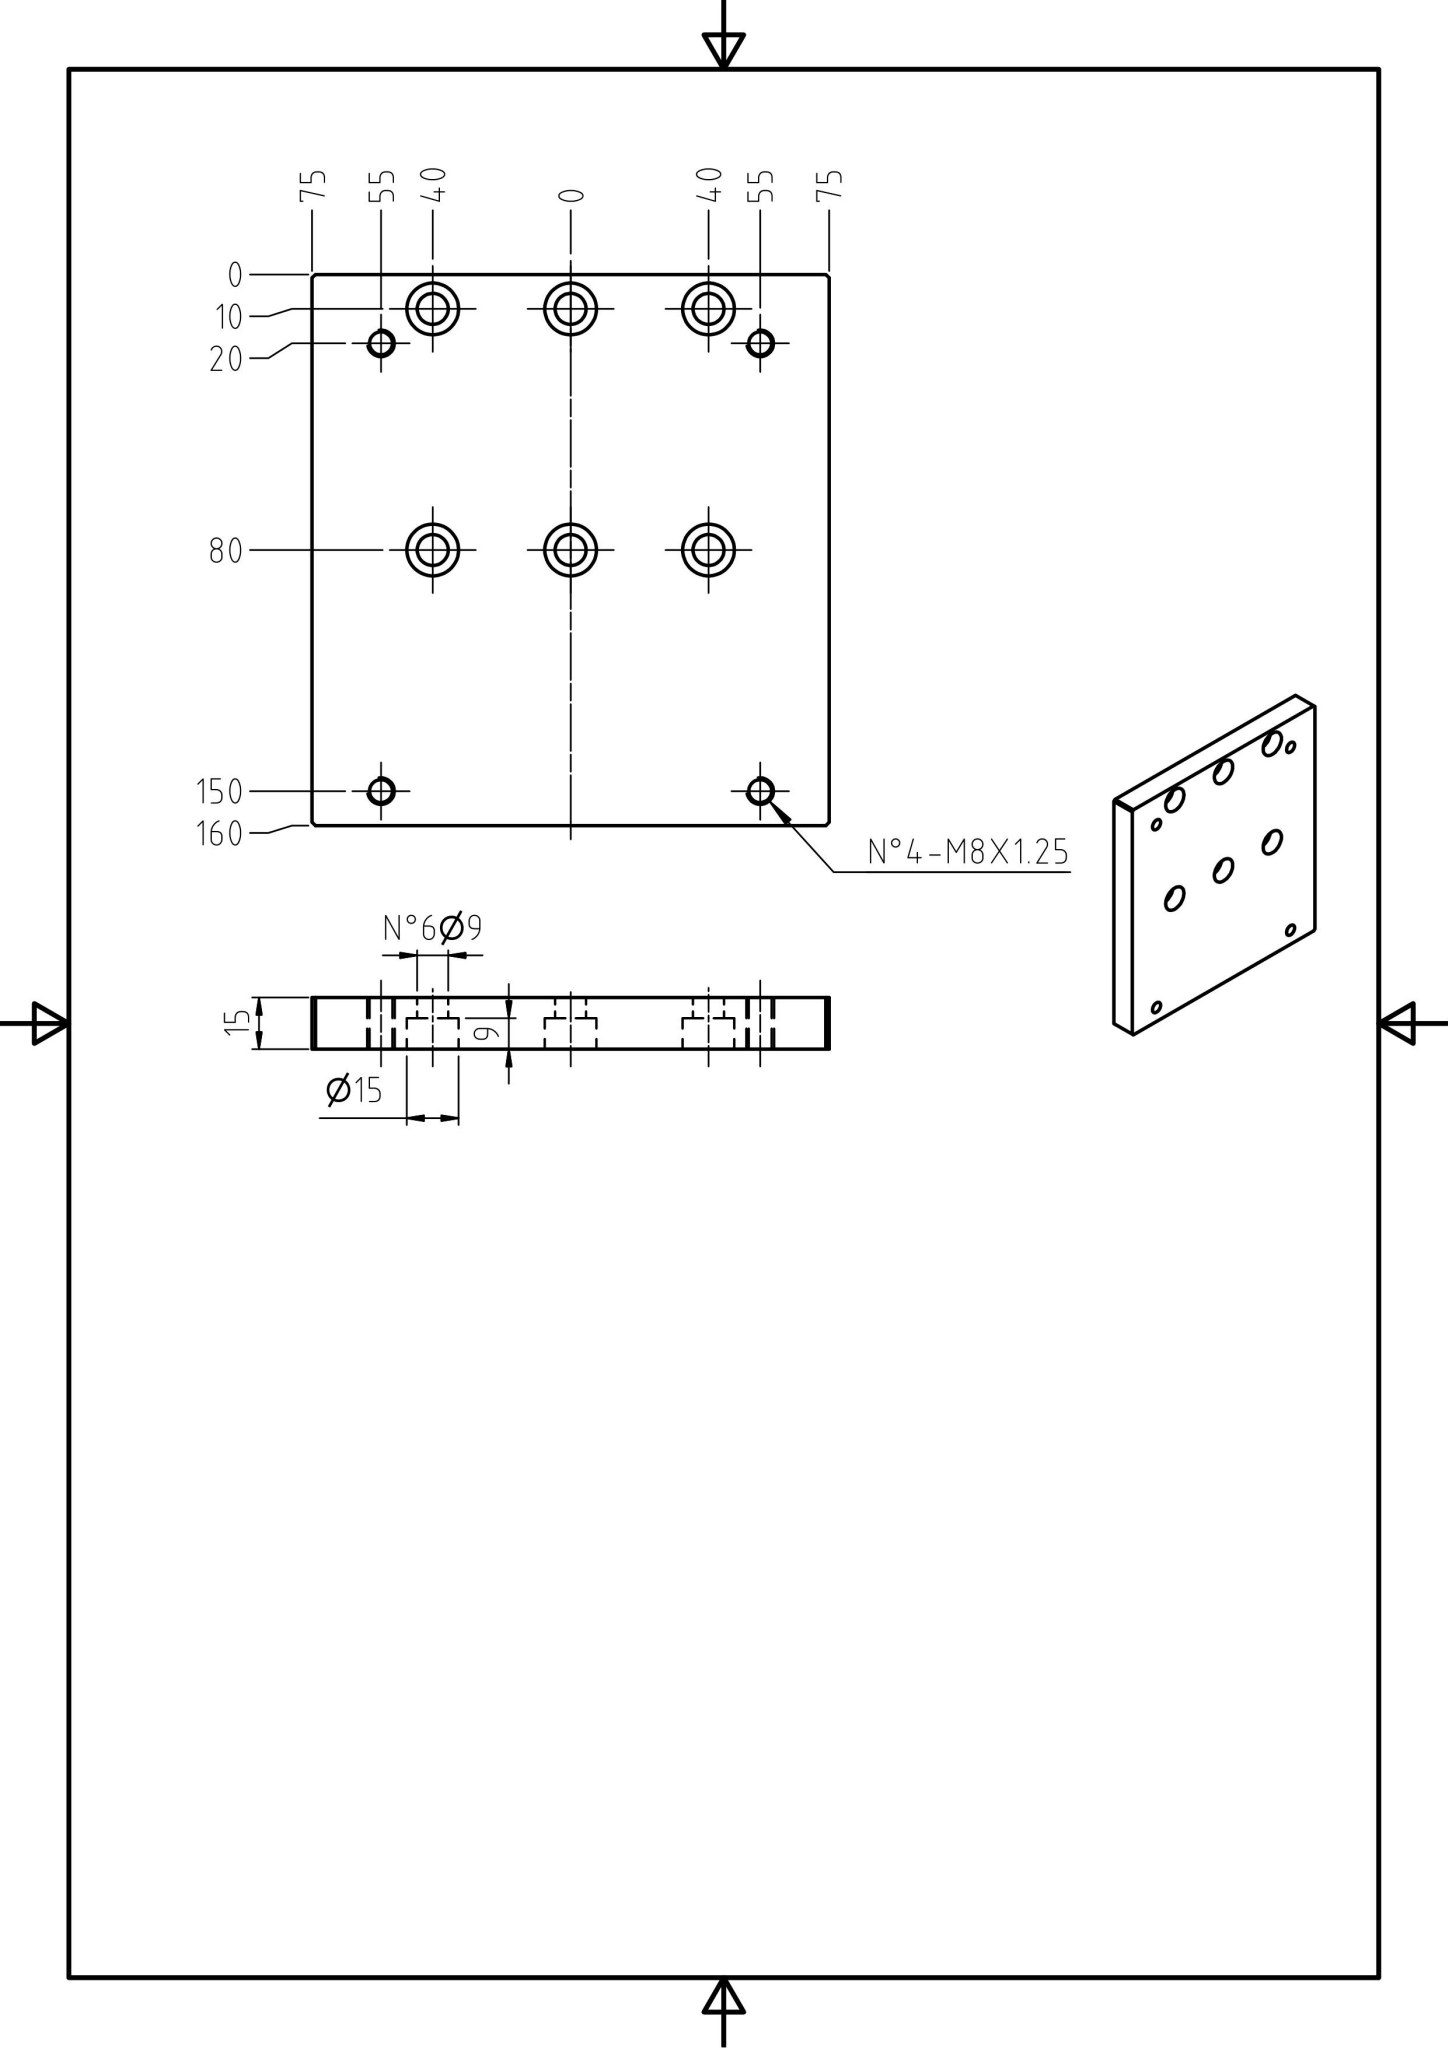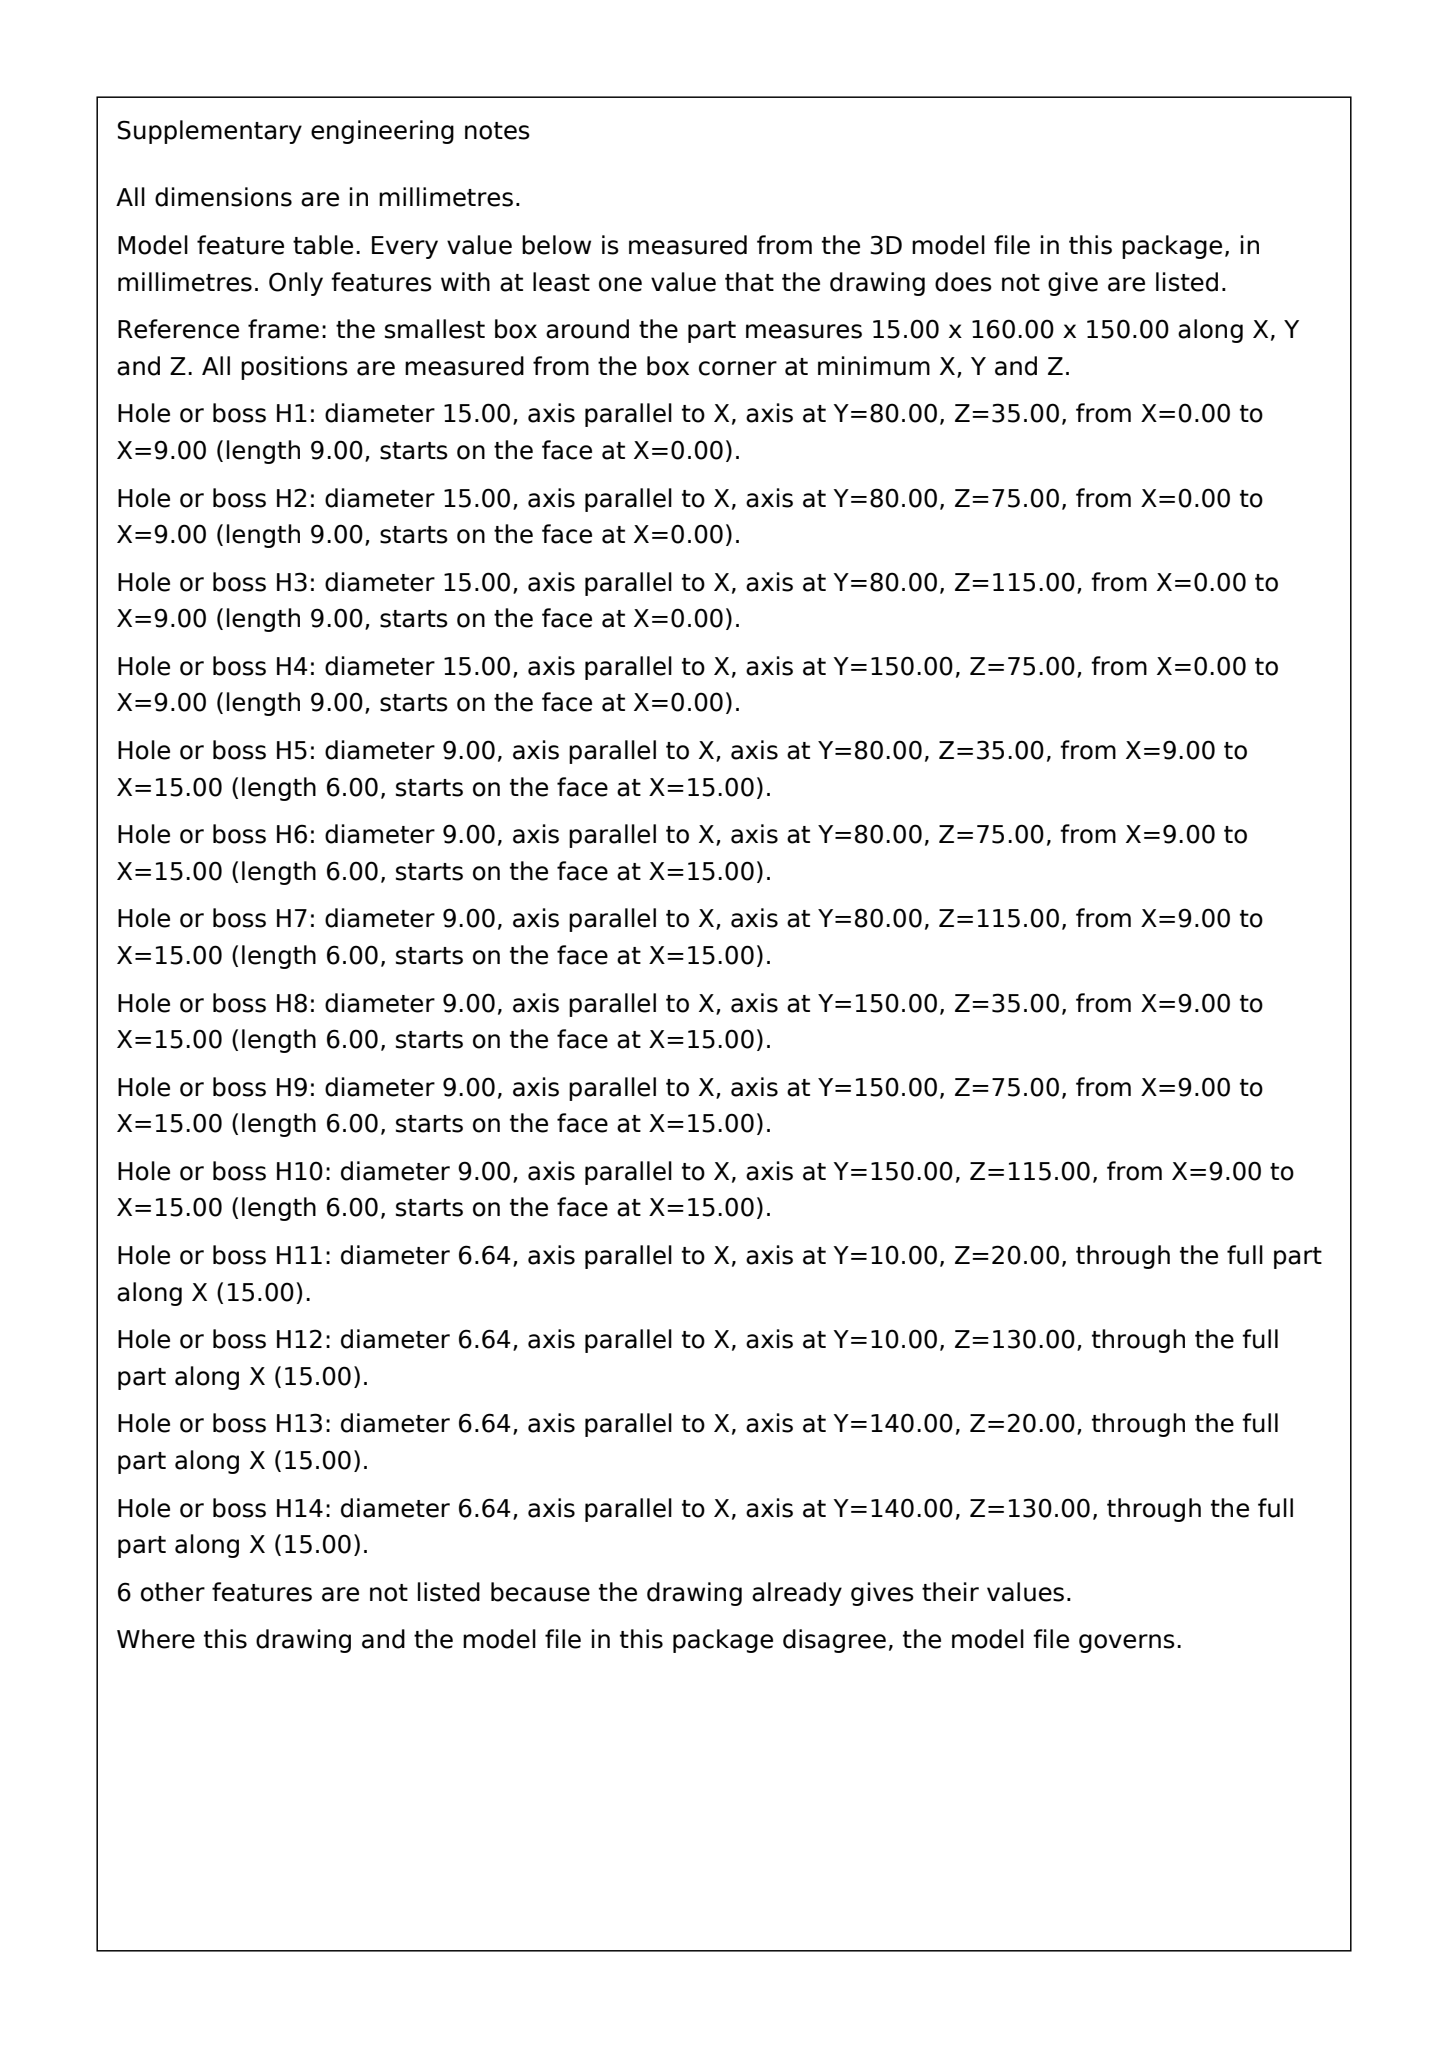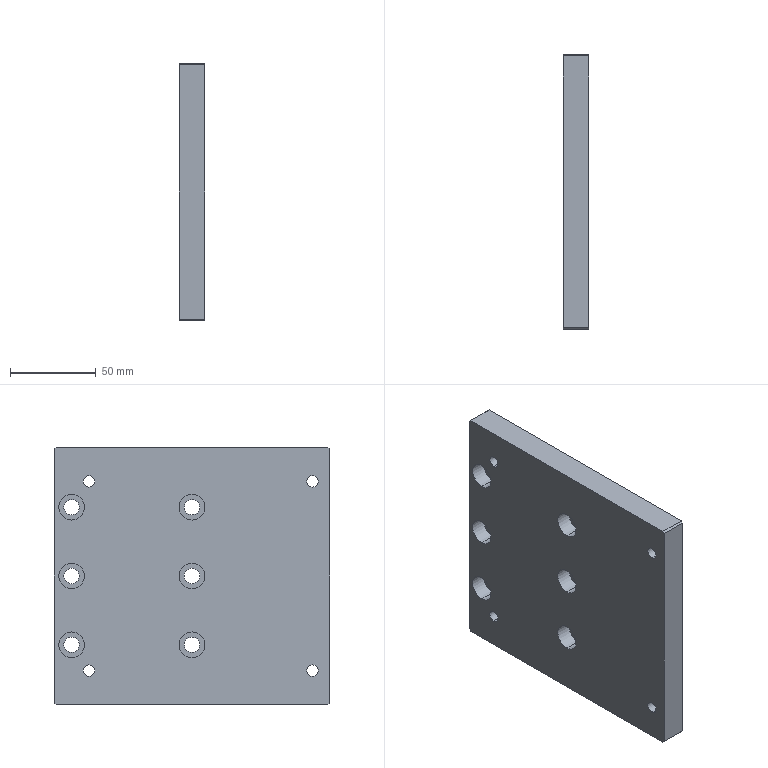Part | SolidWorks | mm | 1 solid | 48 faces | box 15 x 160 x 150 mm | volume 346055 mm3 | cylinder 32 | plane 16 | commonest cylinder face diameters 9 x12 15 x12 6.647 x8